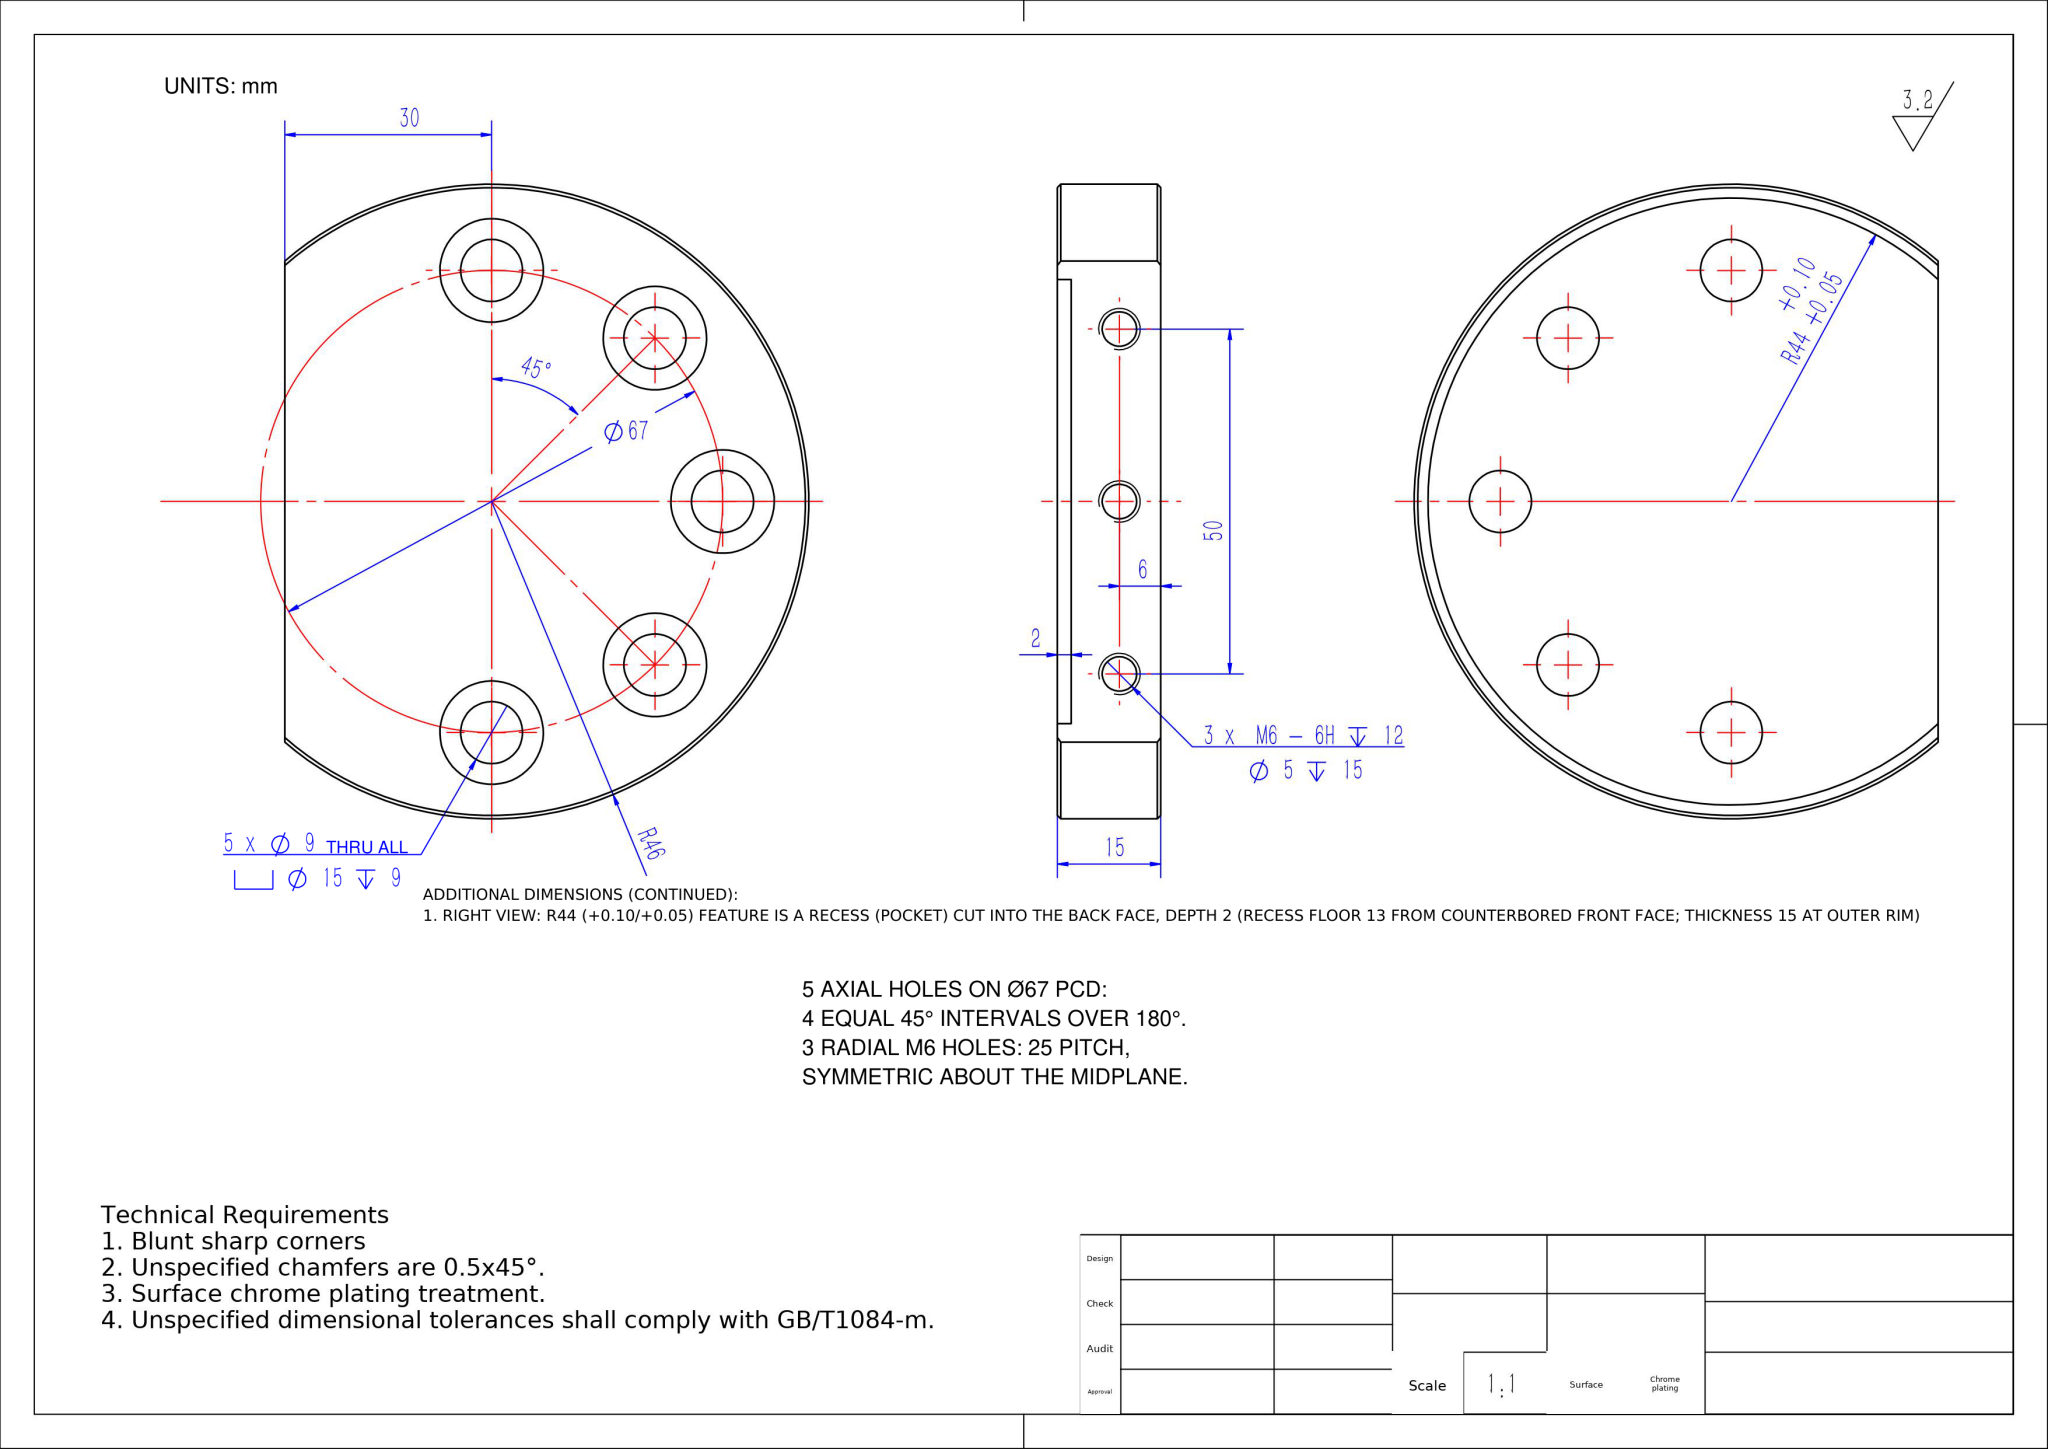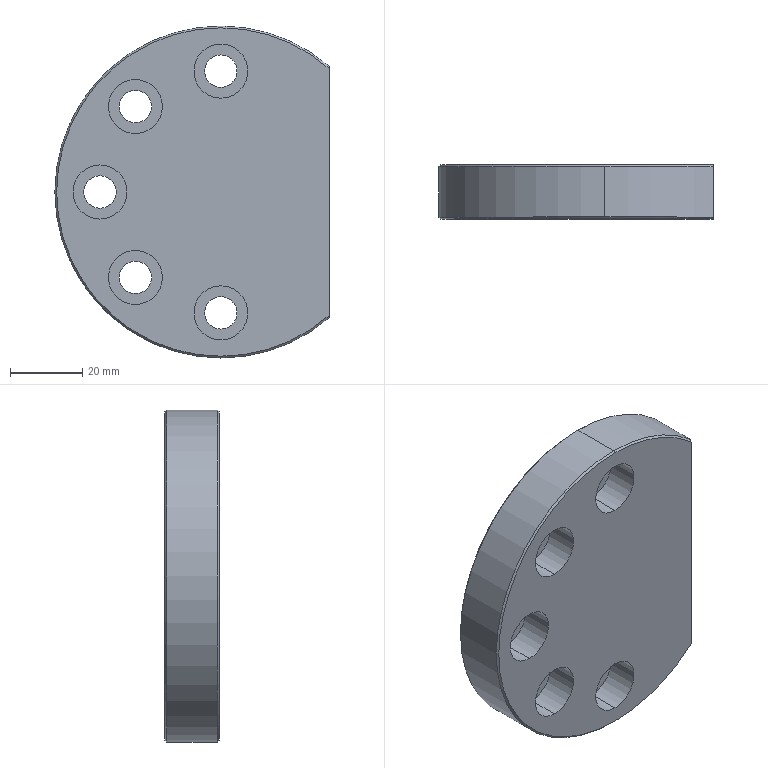Part | NX | mm | 1 solid | 53 faces | box 76 x 15 x 92 mm | volume 66991 mm3 | cylinder 32 | cone 12 | plane 9 | commonest cylinder face diameters 15 x10 9 x10 5 x6 88 x3 92 x3